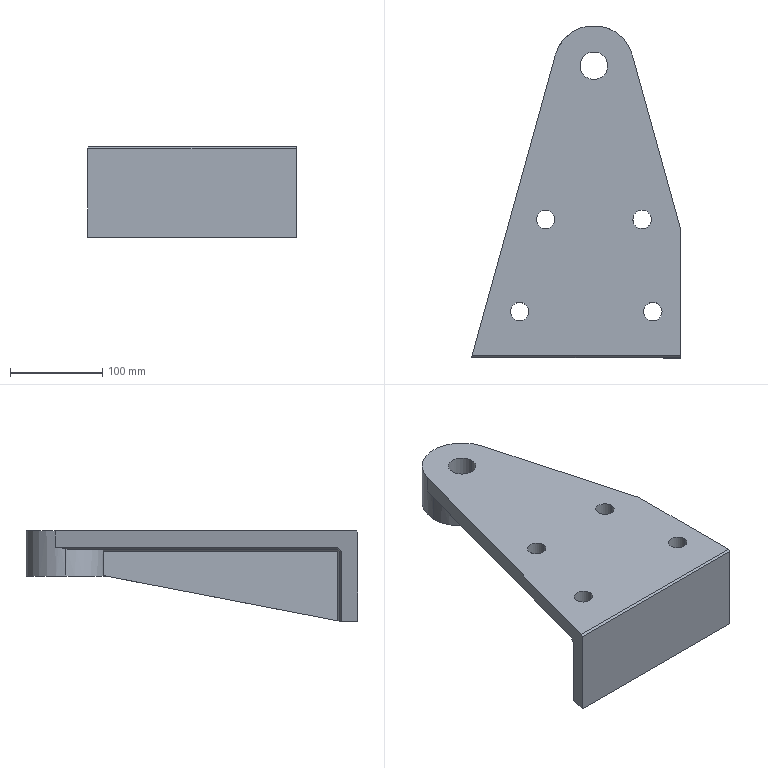Component | SolidWorks | SupportBase3-4 | 1 solid | 40 faces | volume 2001580 mm3 | plane 26 | cylinder 13 | spline 1 | commonest cylinder face diameters 20 x8 86.865 x3 30 x2 | material 45